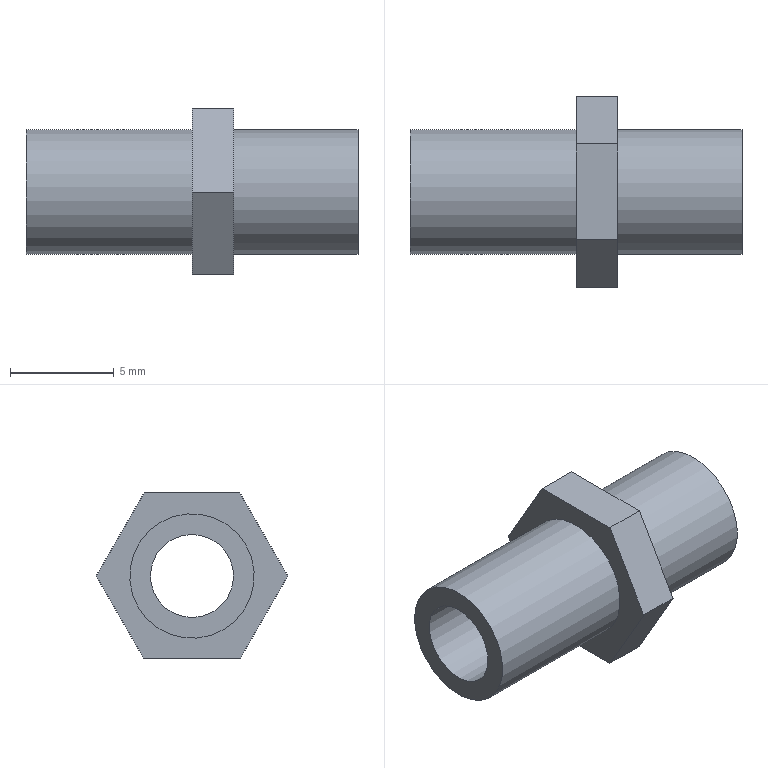Component | NX | PIPE | 1 solid | 13 faces | box 16 x 9.24 x 8 mm | volume 306 mm3 | plane 10 | cylinder 3 | commonest cylinder face diameters 6 x2 4 x1
STEP:
#1=CARTESIAN_POINT('',(0.,0.,0.));
#2=DIRECTION('',(0.,0.,1.));
#3=DIRECTION('',(1.,0.,0.));
#4=AXIS2_PLACEMENT_3D('',#1,#2,#3);
#5=CARTESIAN_POINT('',(-40.,-13.5,42.232));
#6=VERTEX_POINT('',#5);
#7=CARTESIAN_POINT('',(-40.,-14.5,40.5));
#8=DIRECTION('',(1.,0.,0.));
#9=DIRECTION('',(0.,0.5,0.866));
#10=AXIS2_PLACEMENT_3D('',#7,#8,#9);
#11=CIRCLE('',#10,2.);
#12=CARTESIAN_POINT('',(-40.,-14.5,40.5));
#13=DIRECTION('',(-1.,0.,0.));
#14=DIRECTION('',(0.,0.5,0.866));
#15=AXIS2_PLACEMENT_3D('',#12,#13,#14);
#16=PLANE('',#15);
#17=CARTESIAN_POINT('',(2.,-0.));
#18=CARTESIAN_POINT('',(2.,-3.464));
#19=CARTESIAN_POINT('',(-1.,-1.732));
#20=CARTESIAN_POINT('',(-4.,0.));
#21=CARTESIAN_POINT('',(-1.,1.732));
#22=CARTESIAN_POINT('',(2.,3.464));
#23=CARTESIAN_POINT('',(2.,-0.));
#24=(BOUNDED_CURVE()B_SPLINE_CURVE(2,(#17,#18,#19,#20,#21,#22,#23),.UNSPECIFIED.,.T.,.F.)B_SPLINE_CURVE_WITH_KNOTS((1,2,2,2,2,1),(-2.094,0.,2.094,4.189,6.283,8.378),.UNSPECIFIED.)CURVE()GEOMETRIC_REPRESENTATION_ITEM()RATIONAL_B_SPLINE_CURVE((1.,0.5,1.,0.5,1.,0.5,1.))REPRESENTATION_ITEM(''));
#25=(GEOMETRIC_REPRESENTATION_CONTEXT(2)PARAMETRIC_REPRESENTATION_CONTEXT()REPRESENTATION_CONTEXT('',''));
#26=DEFINITIONAL_REPRESENTATION('',(#24),#25);
#27=PCURVE('',#16,#26);
#28=CARTESIAN_POINT('',(-20.,-14.5,40.5));
#29=DIRECTION('',(-1.,0.,0.));
#30=DIRECTION('',(0.,0.5,0.866));
#31=AXIS2_PLACEMENT_3D('',#28,#29,#30);
#32=CYLINDRICAL_SURFACE('',#31,2.);
#33=CARTESIAN_POINT('',(6.283,20.));
#34=DIRECTION('',(-1.,0.));
#35=VECTOR('',#34,1.);
#36=LINE('',#33,#35);
#37=(GEOMETRIC_REPRESENTATION_CONTEXT(2)PARAMETRIC_REPRESENTATION_CONTEXT()REPRESENTATION_CONTEXT('',''));
#38=DEFINITIONAL_REPRESENTATION('',(#36),#37);
#39=PCURVE('',#32,#38);
#40=SURFACE_CURVE('',#11,(#27,#39),.PCURVE_S1.);
#41=EDGE_CURVE('',#6,#6,#40,.T.);
#42=ORIENTED_EDGE('',*,*,#41,.T.);
#43=EDGE_LOOP('',(#42));
#44=FACE_BOUND('',#43,.T.);
#45=CARTESIAN_POINT('',(-40.,-16.,37.902));
#46=VERTEX_POINT('',#45);
#47=CARTESIAN_POINT('',(-40.,-14.5,40.5));
#48=DIRECTION('',(1.,0.,0.));
#49=DIRECTION('',(0.,-0.5,-0.866));
#50=AXIS2_PLACEMENT_3D('',#47,#48,#49);
#51=CIRCLE('',#50,3.);
#52=CARTESIAN_POINT('',(-3.,-0.));
#53=CARTESIAN_POINT('',(-3.,5.196));
#54=CARTESIAN_POINT('',(1.5,2.598));
#55=CARTESIAN_POINT('',(6.,0.));
#56=CARTESIAN_POINT('',(1.5,-2.598));
#57=CARTESIAN_POINT('',(-3.,-5.196));
#58=CARTESIAN_POINT('',(-3.,-0.));
#59=(BOUNDED_CURVE()B_SPLINE_CURVE(2,(#52,#53,#54,#55,#56,#57,#58),.UNSPECIFIED.,.T.,.F.)B_SPLINE_CURVE_WITH_KNOTS((1,2,2,2,2,1),(-2.094,0.,2.094,4.189,6.283,8.378),.UNSPECIFIED.)CURVE()GEOMETRIC_REPRESENTATION_ITEM()RATIONAL_B_SPLINE_CURVE((1.,0.5,1.,0.5,1.,0.5,1.))REPRESENTATION_ITEM(''));
#60=(GEOMETRIC_REPRESENTATION_CONTEXT(2)PARAMETRIC_REPRESENTATION_CONTEXT()REPRESENTATION_CONTEXT('',''));
#61=DEFINITIONAL_REPRESENTATION('',(#59),#60);
#62=PCURVE('',#16,#61);
#63=CARTESIAN_POINT('',(-40.,-14.5,40.5));
#64=DIRECTION('',(1.,0.,0.));
#65=DIRECTION('',(0.,-0.5,-0.866));
#66=AXIS2_PLACEMENT_3D('',#63,#64,#65);
#67=CYLINDRICAL_SURFACE('',#66,3.);
#68=CARTESIAN_POINT('',(0.,0.));
#69=DIRECTION('',(1.,0.));
#70=VECTOR('',#69,1.);
#71=LINE('',#68,#70);
#72=(GEOMETRIC_REPRESENTATION_CONTEXT(2)PARAMETRIC_REPRESENTATION_CONTEXT()REPRESENTATION_CONTEXT('',''));
#73=DEFINITIONAL_REPRESENTATION('',(#71),#72);
#74=PCURVE('',#67,#73);
#75=SURFACE_CURVE('',#51,(#62,#74),.PCURVE_S1.);
#76=EDGE_CURVE('',#46,#46,#75,.T.);
#77=ORIENTED_EDGE('',*,*,#76,.F.);
#78=EDGE_LOOP('',(#77));
#79=FACE_BOUND('',#78,.T.);
#80=ADVANCED_FACE('',(#44,#79),#16,.T.);
#81=CARTESIAN_POINT('',(-32.,-16.,37.902));
#82=VERTEX_POINT('',#81);
#83=CARTESIAN_POINT('',(-32.,-14.5,40.5));
#84=DIRECTION('',(-1.,0.,0.));
#85=DIRECTION('',(0.,-0.5,-0.866));
#86=AXIS2_PLACEMENT_3D('',#83,#84,#85);
#87=CIRCLE('',#86,3.);
#88=CARTESIAN_POINT('',(6.283,8.));
#89=DIRECTION('',(-1.,0.));
#90=VECTOR('',#89,1.);
#91=LINE('',#88,#90);
#92=(GEOMETRIC_REPRESENTATION_CONTEXT(2)PARAMETRIC_REPRESENTATION_CONTEXT()REPRESENTATION_CONTEXT('',''));
#93=DEFINITIONAL_REPRESENTATION('',(#91),#92);
#94=PCURVE('',#67,#93);
#95=CARTESIAN_POINT('',(-32.,-14.5,40.5));
#96=DIRECTION('',(1.,0.,0.));
#97=DIRECTION('',(0.,-0.5,-0.866));
#98=AXIS2_PLACEMENT_3D('',#95,#96,#97);
#99=PLANE('',#98);
#100=CARTESIAN_POINT('',(3.,-0.));
#101=CARTESIAN_POINT('',(3.,-5.196));
#102=CARTESIAN_POINT('',(-1.5,-2.598));
#103=CARTESIAN_POINT('',(-6.,0.));
#104=CARTESIAN_POINT('',(-1.5,2.598));
#105=CARTESIAN_POINT('',(3.,5.196));
#106=CARTESIAN_POINT('',(3.,-0.));
#107=(BOUNDED_CURVE()B_SPLINE_CURVE(2,(#100,#101,#102,#103,#104,#105,#106),.UNSPECIFIED.,.T.,.F.)B_SPLINE_CURVE_WITH_KNOTS((1,2,2,2,2,1),(-2.094,0.,2.094,4.189,6.283,8.378),.UNSPECIFIED.)CURVE()GEOMETRIC_REPRESENTATION_ITEM()RATIONAL_B_SPLINE_CURVE((1.,0.5,1.,0.5,1.,0.5,1.))REPRESENTATION_ITEM(''));
#108=(GEOMETRIC_REPRESENTATION_CONTEXT(2)PARAMETRIC_REPRESENTATION_CONTEXT()REPRESENTATION_CONTEXT('',''));
#109=DEFINITIONAL_REPRESENTATION('',(#107),#108);
#110=PCURVE('',#99,#109);
#111=SURFACE_CURVE('',#87,(#94,#110),.PCURVE_S1.);
#112=EDGE_CURVE('',#82,#82,#111,.T.);
#113=ORIENTED_EDGE('',*,*,#112,.T.);
#114=CARTESIAN_POINT('',(-40.,-16.,37.902));
#115=CARTESIAN_POINT('',(-32.,-16.,37.902));
#116=B_SPLINE_CURVE_WITH_KNOTS('',1,(#114,#115),.UNSPECIFIED.,.F.,.F.,(2,2),(0.,8.),.PIECEWISE_BEZIER_KNOTS.);
#117=CARTESIAN_POINT('',(0.,0.));
#118=DIRECTION('',(0.,1.));
#119=VECTOR('',#118,1.);
#120=LINE('',#117,#119);
#121=(GEOMETRIC_REPRESENTATION_CONTEXT(2)PARAMETRIC_REPRESENTATION_CONTEXT()REPRESENTATION_CONTEXT('',''));
#122=DEFINITIONAL_REPRESENTATION('',(#120),#121);
#123=PCURVE('',#67,#122);
#124=CARTESIAN_POINT('',(6.283,0.));
#125=DIRECTION('',(0.,1.));
#126=VECTOR('',#125,1.);
#127=LINE('',#124,#126);
#128=(GEOMETRIC_REPRESENTATION_CONTEXT(2)PARAMETRIC_REPRESENTATION_CONTEXT()REPRESENTATION_CONTEXT('',''));
#129=DEFINITIONAL_REPRESENTATION('',(#127),#128);
#130=PCURVE('',#67,#129);
#131=SEAM_CURVE('',#116,(#123,#130),.PCURVE_S1.);
#132=EDGE_CURVE('',#46,#82,#131,.T.);
#133=ORIENTED_EDGE('',*,*,#132,.F.);
#134=ORIENTED_EDGE('',*,*,#76,.T.);
#135=ORIENTED_EDGE('',*,*,#132,.T.);
#136=EDGE_LOOP('',(#113,#133,#134,#135));
#137=FACE_BOUND('',#136,.T.);
#138=ADVANCED_FACE('',(#137),#67,.T.);
#139=CARTESIAN_POINT('',(-32.,-12.191,44.5));
#140=VERTEX_POINT('',#139);
#141=CARTESIAN_POINT('',(-32.,-16.809,44.5));
#142=VERTEX_POINT('',#141);
#143=CARTESIAN_POINT('',(-32.,-12.191,44.5));
#144=DIRECTION('',(0.,-1.,-0.));
#145=VECTOR('',#144,1.);
#146=LINE('',#143,#145);
#147=CARTESIAN_POINT('',(-30.,-12.191,44.5));
#148=DIRECTION('',(0.,0.,-1.));
#149=DIRECTION('',(0.,1.,0.));
#150=AXIS2_PLACEMENT_3D('',#147,#148,#149);
#151=PLANE('',#150);
#152=CARTESIAN_POINT('',(0.,-2.));
#153=DIRECTION('',(-1.,0.));
#154=VECTOR('',#153,1.);
#155=LINE('',#152,#154);
#156=(GEOMETRIC_REPRESENTATION_CONTEXT(2)PARAMETRIC_REPRESENTATION_CONTEXT()REPRESENTATION_CONTEXT('',''));
#157=DEFINITIONAL_REPRESENTATION('',(#155),#156);
#158=PCURVE('',#151,#157);
#159=CARTESIAN_POINT('',(-4.619,-0.));
#160=DIRECTION('',(0.5,-0.866));
#161=VECTOR('',#160,1.);
#162=LINE('',#159,#161);
#163=(GEOMETRIC_REPRESENTATION_CONTEXT(2)PARAMETRIC_REPRESENTATION_CONTEXT()REPRESENTATION_CONTEXT('',''));
#164=DEFINITIONAL_REPRESENTATION('',(#162),#163);
#165=PCURVE('',#99,#164);
#166=SURFACE_CURVE('',#146,(#158,#165),.PCURVE_S1.);
#167=EDGE_CURVE('',#140,#142,#166,.T.);
#168=ORIENTED_EDGE('',*,*,#167,.T.);
#169=CARTESIAN_POINT('',(-30.,-16.809,44.5));
#170=VERTEX_POINT('',#169);
#171=CARTESIAN_POINT('',(-30.,-16.809,44.5));
#172=DIRECTION('',(-1.,0.,0.));
#173=VECTOR('',#172,1.);
#174=LINE('',#171,#173);
#175=CARTESIAN_POINT('',(-4.619,0.));
#176=DIRECTION('',(0.,-1.));
#177=VECTOR('',#176,1.);
#178=LINE('',#175,#177);
#179=(GEOMETRIC_REPRESENTATION_CONTEXT(2)PARAMETRIC_REPRESENTATION_CONTEXT()REPRESENTATION_CONTEXT('',''));
#180=DEFINITIONAL_REPRESENTATION('',(#178),#179);
#181=PCURVE('',#151,#180);
#182=CARTESIAN_POINT('',(-30.,-16.809,44.5));
#183=DIRECTION('',(0.,0.866,-0.5));
#184=DIRECTION('',(0.,0.5,0.866));
#185=AXIS2_PLACEMENT_3D('',#182,#183,#184);
#186=PLANE('',#185);
#187=CARTESIAN_POINT('',(0.,0.));
#188=DIRECTION('',(0.,-1.));
#189=VECTOR('',#188,1.);
#190=LINE('',#187,#189);
#191=(GEOMETRIC_REPRESENTATION_CONTEXT(2)PARAMETRIC_REPRESENTATION_CONTEXT()REPRESENTATION_CONTEXT('',''));
#192=DEFINITIONAL_REPRESENTATION('',(#190),#191);
#193=PCURVE('',#186,#192);
#194=SURFACE_CURVE('',#174,(#181,#193),.PCURVE_S1.);
#195=EDGE_CURVE('',#170,#142,#194,.T.);
#196=ORIENTED_EDGE('',*,*,#195,.F.);
#197=CARTESIAN_POINT('',(-30.,-12.191,44.5));
#198=VERTEX_POINT('',#197);
#199=CARTESIAN_POINT('',(-30.,-12.191,44.5));
#200=DIRECTION('',(0.,-1.,-0.));
#201=VECTOR('',#200,1.);
#202=LINE('',#199,#201);
#203=CARTESIAN_POINT('',(0.,0.));
#204=DIRECTION('',(-1.,0.));
#205=VECTOR('',#204,1.);
#206=LINE('',#203,#205);
#207=(GEOMETRIC_REPRESENTATION_CONTEXT(2)PARAMETRIC_REPRESENTATION_CONTEXT()REPRESENTATION_CONTEXT('',''));
#208=DEFINITIONAL_REPRESENTATION('',(#206),#207);
#209=PCURVE('',#151,#208);
#210=CARTESIAN_POINT('',(-30.,-14.5,40.5));
#211=DIRECTION('',(1.,0.,0.));
#212=DIRECTION('',(0.,-0.5,-0.866));
#213=AXIS2_PLACEMENT_3D('',#210,#211,#212);
#214=PLANE('',#213);
#215=CARTESIAN_POINT('',(-4.619,-0.));
#216=DIRECTION('',(0.5,-0.866));
#217=VECTOR('',#216,1.);
#218=LINE('',#215,#217);
#219=(GEOMETRIC_REPRESENTATION_CONTEXT(2)PARAMETRIC_REPRESENTATION_CONTEXT()REPRESENTATION_CONTEXT('',''));
#220=DEFINITIONAL_REPRESENTATION('',(#218),#219);
#221=PCURVE('',#214,#220);
#222=SURFACE_CURVE('',#202,(#209,#221),.PCURVE_S1.);
#223=EDGE_CURVE('',#198,#170,#222,.T.);
#224=ORIENTED_EDGE('',*,*,#223,.F.);
#225=CARTESIAN_POINT('',(-30.,-12.191,44.5));
#226=DIRECTION('',(-1.,0.,0.));
#227=VECTOR('',#226,1.);
#228=LINE('',#225,#227);
#229=CARTESIAN_POINT('',(0.,0.));
#230=DIRECTION('',(0.,-1.));
#231=VECTOR('',#230,1.);
#232=LINE('',#229,#231);
#233=(GEOMETRIC_REPRESENTATION_CONTEXT(2)PARAMETRIC_REPRESENTATION_CONTEXT()REPRESENTATION_CONTEXT('',''));
#234=DEFINITIONAL_REPRESENTATION('',(#232),#233);
#235=PCURVE('',#151,#234);
#236=CARTESIAN_POINT('',(-30.,-9.881,40.5));
#237=DIRECTION('',(0.,-0.866,-0.5));
#238=DIRECTION('',(0.,0.5,-0.866));
#239=AXIS2_PLACEMENT_3D('',#236,#237,#238);
#240=PLANE('',#239);
#241=CARTESIAN_POINT('',(-4.619,0.));
#242=DIRECTION('',(0.,-1.));
#243=VECTOR('',#242,1.);
#244=LINE('',#241,#243);
#245=(GEOMETRIC_REPRESENTATION_CONTEXT(2)PARAMETRIC_REPRESENTATION_CONTEXT()REPRESENTATION_CONTEXT('',''));
#246=DEFINITIONAL_REPRESENTATION('',(#244),#245);
#247=PCURVE('',#240,#246);
#248=SURFACE_CURVE('',#228,(#235,#247),.PCURVE_S1.);
#249=EDGE_CURVE('',#198,#140,#248,.T.);
#250=ORIENTED_EDGE('',*,*,#249,.T.);
#251=EDGE_LOOP('',(#168,#196,#224,#250));
#252=FACE_BOUND('',#251,.T.);
#253=ADVANCED_FACE('',(#252),#151,.F.);
#254=CARTESIAN_POINT('',(-32.,-19.119,40.5));
#255=VERTEX_POINT('',#254);
#256=CARTESIAN_POINT('',(-32.,-16.809,44.5));
#257=DIRECTION('',(0.,-0.5,-0.866));
#258=VECTOR('',#257,1.);
#259=LINE('',#256,#258);
#260=CARTESIAN_POINT('',(0.,-2.));
#261=DIRECTION('',(-1.,0.));
#262=VECTOR('',#261,1.);
#263=LINE('',#260,#262);
#264=(GEOMETRIC_REPRESENTATION_CONTEXT(2)PARAMETRIC_REPRESENTATION_CONTEXT()REPRESENTATION_CONTEXT('',''));
#265=DEFINITIONAL_REPRESENTATION('',(#263),#264);
#266=PCURVE('',#186,#265);
#267=CARTESIAN_POINT('',(-2.309,-4.));
#268=DIRECTION('',(1.,0.));
#269=VECTOR('',#268,1.);
#270=LINE('',#267,#269);
#271=(GEOMETRIC_REPRESENTATION_CONTEXT(2)PARAMETRIC_REPRESENTATION_CONTEXT()REPRESENTATION_CONTEXT('',''));
#272=DEFINITIONAL_REPRESENTATION('',(#270),#271);
#273=PCURVE('',#99,#272);
#274=SURFACE_CURVE('',#259,(#266,#273),.PCURVE_S1.);
#275=EDGE_CURVE('',#142,#255,#274,.T.);
#276=ORIENTED_EDGE('',*,*,#275,.T.);
#277=CARTESIAN_POINT('',(-30.,-19.119,40.5));
#278=VERTEX_POINT('',#277);
#279=CARTESIAN_POINT('',(-30.,-19.119,40.5));
#280=DIRECTION('',(-1.,0.,0.));
#281=VECTOR('',#280,1.);
#282=LINE('',#279,#281);
#283=CARTESIAN_POINT('',(-4.619,0.));
#284=DIRECTION('',(0.,-1.));
#285=VECTOR('',#284,1.);
#286=LINE('',#283,#285);
#287=(GEOMETRIC_REPRESENTATION_CONTEXT(2)PARAMETRIC_REPRESENTATION_CONTEXT()REPRESENTATION_CONTEXT('',''));
#288=DEFINITIONAL_REPRESENTATION('',(#286),#287);
#289=PCURVE('',#186,#288);
#290=CARTESIAN_POINT('',(-30.,-19.119,40.5));
#291=DIRECTION('',(0.,0.866,0.5));
#292=DIRECTION('',(0.,-0.5,0.866));
#293=AXIS2_PLACEMENT_3D('',#290,#291,#292);
#294=PLANE('',#293);
#295=CARTESIAN_POINT('',(0.,0.));
#296=DIRECTION('',(0.,-1.));
#297=VECTOR('',#296,1.);
#298=LINE('',#295,#297);
#299=(GEOMETRIC_REPRESENTATION_CONTEXT(2)PARAMETRIC_REPRESENTATION_CONTEXT()REPRESENTATION_CONTEXT('',''));
#300=DEFINITIONAL_REPRESENTATION('',(#298),#299);
#301=PCURVE('',#294,#300);
#302=SURFACE_CURVE('',#282,(#289,#301),.PCURVE_S1.);
#303=EDGE_CURVE('',#278,#255,#302,.T.);
#304=ORIENTED_EDGE('',*,*,#303,.F.);
#305=CARTESIAN_POINT('',(-30.,-16.809,44.5));
#306=DIRECTION('',(0.,-0.5,-0.866));
#307=VECTOR('',#306,1.);
#308=LINE('',#305,#307);
#309=CARTESIAN_POINT('',(0.,0.));
#310=DIRECTION('',(-1.,0.));
#311=VECTOR('',#310,1.);
#312=LINE('',#309,#311);
#313=(GEOMETRIC_REPRESENTATION_CONTEXT(2)PARAMETRIC_REPRESENTATION_CONTEXT()REPRESENTATION_CONTEXT('',''));
#314=DEFINITIONAL_REPRESENTATION('',(#312),#313);
#315=PCURVE('',#186,#314);
#316=CARTESIAN_POINT('',(-2.309,-4.));
#317=DIRECTION('',(1.,0.));
#318=VECTOR('',#317,1.);
#319=LINE('',#316,#318);
#320=(GEOMETRIC_REPRESENTATION_CONTEXT(2)PARAMETRIC_REPRESENTATION_CONTEXT()REPRESENTATION_CONTEXT('',''));
#321=DEFINITIONAL_REPRESENTATION('',(#319),#320);
#322=PCURVE('',#214,#321);
#323=SURFACE_CURVE('',#308,(#315,#322),.PCURVE_S1.);
#324=EDGE_CURVE('',#170,#278,#323,.T.);
#325=ORIENTED_EDGE('',*,*,#324,.F.);
#326=ORIENTED_EDGE('',*,*,#195,.T.);
#327=EDGE_LOOP('',(#276,#304,#325,#326));
#328=FACE_BOUND('',#327,.T.);
#329=ADVANCED_FACE('',(#328),#186,.F.);
#330=CARTESIAN_POINT('',(-32.,-16.809,36.5));
#331=VERTEX_POINT('',#330);
#332=CARTESIAN_POINT('',(-32.,-19.119,40.5));
#333=DIRECTION('',(0.,0.5,-0.866));
#334=VECTOR('',#333,1.);
#335=LINE('',#332,#334);
#336=CARTESIAN_POINT('',(0.,-2.));
#337=DIRECTION('',(-1.,0.));
#338=VECTOR('',#337,1.);
#339=LINE('',#336,#338);
#340=(GEOMETRIC_REPRESENTATION_CONTEXT(2)PARAMETRIC_REPRESENTATION_CONTEXT()REPRESENTATION_CONTEXT('',''));
#341=DEFINITIONAL_REPRESENTATION('',(#339),#340);
#342=PCURVE('',#294,#341);
#343=CARTESIAN_POINT('',(2.309,-4.));
#344=DIRECTION('',(0.5,0.866));
#345=VECTOR('',#344,1.);
#346=LINE('',#343,#345);
#347=(GEOMETRIC_REPRESENTATION_CONTEXT(2)PARAMETRIC_REPRESENTATION_CONTEXT()REPRESENTATION_CONTEXT('',''));
#348=DEFINITIONAL_REPRESENTATION('',(#346),#347);
#349=PCURVE('',#99,#348);
#350=SURFACE_CURVE('',#335,(#342,#349),.PCURVE_S1.);
#351=EDGE_CURVE('',#255,#331,#350,.T.);
#352=ORIENTED_EDGE('',*,*,#351,.T.);
#353=CARTESIAN_POINT('',(-30.,-16.809,36.5));
#354=VERTEX_POINT('',#353);
#355=CARTESIAN_POINT('',(-30.,-16.809,36.5));
#356=DIRECTION('',(-1.,0.,0.));
#357=VECTOR('',#356,1.);
#358=LINE('',#355,#357);
#359=CARTESIAN_POINT('',(-4.619,0.));
#360=DIRECTION('',(0.,-1.));
#361=VECTOR('',#360,1.);
#362=LINE('',#359,#361);
#363=(GEOMETRIC_REPRESENTATION_CONTEXT(2)PARAMETRIC_REPRESENTATION_CONTEXT()REPRESENTATION_CONTEXT('',''));
#364=DEFINITIONAL_REPRESENTATION('',(#362),#363);
#365=PCURVE('',#294,#364);
#366=CARTESIAN_POINT('',(-30.,-16.809,36.5));
#367=DIRECTION('',(0.,-0.,1.));
#368=DIRECTION('',(0.,-1.,-0.));
#369=AXIS2_PLACEMENT_3D('',#366,#367,#368);
#370=PLANE('',#369);
#371=CARTESIAN_POINT('',(0.,0.));
#372=DIRECTION('',(0.,-1.));
#373=VECTOR('',#372,1.);
#374=LINE('',#371,#373);
#375=(GEOMETRIC_REPRESENTATION_CONTEXT(2)PARAMETRIC_REPRESENTATION_CONTEXT()REPRESENTATION_CONTEXT('',''));
#376=DEFINITIONAL_REPRESENTATION('',(#374),#375);
#377=PCURVE('',#370,#376);
#378=SURFACE_CURVE('',#358,(#365,#377),.PCURVE_S1.);
#379=EDGE_CURVE('',#354,#331,#378,.T.);
#380=ORIENTED_EDGE('',*,*,#379,.F.);
#381=CARTESIAN_POINT('',(-30.,-19.119,40.5));
#382=DIRECTION('',(0.,0.5,-0.866));
#383=VECTOR('',#382,1.);
#384=LINE('',#381,#383);
#385=CARTESIAN_POINT('',(0.,0.));
#386=DIRECTION('',(-1.,0.));
#387=VECTOR('',#386,1.);
#388=LINE('',#385,#387);
#389=(GEOMETRIC_REPRESENTATION_CONTEXT(2)PARAMETRIC_REPRESENTATION_CONTEXT()REPRESENTATION_CONTEXT('',''));
#390=DEFINITIONAL_REPRESENTATION('',(#388),#389);
#391=PCURVE('',#294,#390);
#392=CARTESIAN_POINT('',(2.309,-4.));
#393=DIRECTION('',(0.5,0.866));
#394=VECTOR('',#393,1.);
#395=LINE('',#392,#394);
#396=(GEOMETRIC_REPRESENTATION_CONTEXT(2)PARAMETRIC_REPRESENTATION_CONTEXT()REPRESENTATION_CONTEXT('',''));
#397=DEFINITIONAL_REPRESENTATION('',(#395),#396);
#398=PCURVE('',#214,#397);
#399=SURFACE_CURVE('',#384,(#391,#398),.PCURVE_S1.);
#400=EDGE_CURVE('',#278,#354,#399,.T.);
#401=ORIENTED_EDGE('',*,*,#400,.F.);
#402=ORIENTED_EDGE('',*,*,#303,.T.);
#403=EDGE_LOOP('',(#352,#380,#401,#402));
#404=FACE_BOUND('',#403,.T.);
#405=ADVANCED_FACE('',(#404),#294,.F.);
#406=CARTESIAN_POINT('',(-32.,-12.191,36.5));
#407=VERTEX_POINT('',#406);
#408=CARTESIAN_POINT('',(-32.,-16.809,36.5));
#409=DIRECTION('',(0.,1.,0.));
#410=VECTOR('',#409,1.);
#411=LINE('',#408,#410);
#412=CARTESIAN_POINT('',(0.,-2.));
#413=DIRECTION('',(-1.,0.));
#414=VECTOR('',#413,1.);
#415=LINE('',#412,#414);
#416=(GEOMETRIC_REPRESENTATION_CONTEXT(2)PARAMETRIC_REPRESENTATION_CONTEXT()REPRESENTATION_CONTEXT('',''));
#417=DEFINITIONAL_REPRESENTATION('',(#415),#416);
#418=PCURVE('',#370,#417);
#419=CARTESIAN_POINT('',(4.619,0.));
#420=DIRECTION('',(-0.5,0.866));
#421=VECTOR('',#420,1.);
#422=LINE('',#419,#421);
#423=(GEOMETRIC_REPRESENTATION_CONTEXT(2)PARAMETRIC_REPRESENTATION_CONTEXT()REPRESENTATION_CONTEXT('',''));
#424=DEFINITIONAL_REPRESENTATION('',(#422),#423);
#425=PCURVE('',#99,#424);
#426=SURFACE_CURVE('',#411,(#418,#425),.PCURVE_S1.);
#427=EDGE_CURVE('',#331,#407,#426,.T.);
#428=ORIENTED_EDGE('',*,*,#427,.T.);
#429=CARTESIAN_POINT('',(-30.,-12.191,36.5));
#430=VERTEX_POINT('',#429);
#431=CARTESIAN_POINT('',(-30.,-12.191,36.5));
#432=DIRECTION('',(-1.,0.,0.));
#433=VECTOR('',#432,1.);
#434=LINE('',#431,#433);
#435=CARTESIAN_POINT('',(-4.619,0.));
#436=DIRECTION('',(0.,-1.));
#437=VECTOR('',#436,1.);
#438=LINE('',#435,#437);
#439=(GEOMETRIC_REPRESENTATION_CONTEXT(2)PARAMETRIC_REPRESENTATION_CONTEXT()REPRESENTATION_CONTEXT('',''));
#440=DEFINITIONAL_REPRESENTATION('',(#438),#439);
#441=PCURVE('',#370,#440);
#442=CARTESIAN_POINT('',(-30.,-12.191,36.5));
#443=DIRECTION('',(0.,-0.866,0.5));
#444=DIRECTION('',(0.,-0.5,-0.866));
#445=AXIS2_PLACEMENT_3D('',#442,#443,#444);
#446=PLANE('',#445);
#447=CARTESIAN_POINT('',(0.,0.));
#448=DIRECTION('',(0.,-1.));
#449=VECTOR('',#448,1.);
#450=LINE('',#447,#449);
#451=(GEOMETRIC_REPRESENTATION_CONTEXT(2)PARAMETRIC_REPRESENTATION_CONTEXT()REPRESENTATION_CONTEXT('',''));
#452=DEFINITIONAL_REPRESENTATION('',(#450),#451);
#453=PCURVE('',#446,#452);
#454=SURFACE_CURVE('',#434,(#441,#453),.PCURVE_S1.);
#455=EDGE_CURVE('',#430,#407,#454,.T.);
#456=ORIENTED_EDGE('',*,*,#455,.F.);
#457=CARTESIAN_POINT('',(-30.,-16.809,36.5));
#458=DIRECTION('',(0.,1.,0.));
#459=VECTOR('',#458,1.);
#460=LINE('',#457,#459);
#461=CARTESIAN_POINT('',(0.,0.));
#462=DIRECTION('',(-1.,0.));
#463=VECTOR('',#462,1.);
#464=LINE('',#461,#463);
#465=(GEOMETRIC_REPRESENTATION_CONTEXT(2)PARAMETRIC_REPRESENTATION_CONTEXT()REPRESENTATION_CONTEXT('',''));
#466=DEFINITIONAL_REPRESENTATION('',(#464),#465);
#467=PCURVE('',#370,#466);
#468=CARTESIAN_POINT('',(4.619,0.));
#469=DIRECTION('',(-0.5,0.866));
#470=VECTOR('',#469,1.);
#471=LINE('',#468,#470);
#472=(GEOMETRIC_REPRESENTATION_CONTEXT(2)PARAMETRIC_REPRESENTATION_CONTEXT()REPRESENTATION_CONTEXT('',''));
#473=DEFINITIONAL_REPRESENTATION('',(#471),#472);
#474=PCURVE('',#214,#473);
#475=SURFACE_CURVE('',#460,(#467,#474),.PCURVE_S1.);
#476=EDGE_CURVE('',#354,#430,#475,.T.);
#477=ORIENTED_EDGE('',*,*,#476,.F.);
#478=ORIENTED_EDGE('',*,*,#379,.T.);
#479=EDGE_LOOP('',(#428,#456,#477,#478));
#480=FACE_BOUND('',#479,.T.);
#481=ADVANCED_FACE('',(#480),#370,.F.);
#482=CARTESIAN_POINT('',(-32.,-9.881,40.5));
#483=VERTEX_POINT('',#482);
#484=CARTESIAN_POINT('',(-32.,-12.191,36.5));
#485=DIRECTION('',(0.,0.5,0.866));
#486=VECTOR('',#485,1.);
#487=LINE('',#484,#486);
#488=CARTESIAN_POINT('',(0.,-2.));
#489=DIRECTION('',(-1.,0.));
#490=VECTOR('',#489,1.);
#491=LINE('',#488,#490);
#492=(GEOMETRIC_REPRESENTATION_CONTEXT(2)PARAMETRIC_REPRESENTATION_CONTEXT()REPRESENTATION_CONTEXT('',''));
#493=DEFINITIONAL_REPRESENTATION('',(#491),#492);
#494=PCURVE('',#446,#493);
#495=CARTESIAN_POINT('',(2.309,4.));
#496=DIRECTION('',(-1.,0.));
#497=VECTOR('',#496,1.);
#498=LINE('',#495,#497);
#499=(GEOMETRIC_REPRESENTATION_CONTEXT(2)PARAMETRIC_REPRESENTATION_CONTEXT()REPRESENTATION_CONTEXT('',''));
#500=DEFINITIONAL_REPRESENTATION('',(#498),#499);
#501=PCURVE('',#99,#500);
#502=SURFACE_CURVE('',#487,(#494,#501),.PCURVE_S1.);
#503=EDGE_CURVE('',#407,#483,#502,.T.);
#504=ORIENTED_EDGE('',*,*,#503,.T.);
#505=CARTESIAN_POINT('',(-30.,-9.881,40.5));
#506=VERTEX_POINT('',#505);
#507=CARTESIAN_POINT('',(-30.,-9.881,40.5));
#508=DIRECTION('',(-1.,0.,0.));
#509=VECTOR('',#508,1.);
#510=LINE('',#507,#509);
#511=CARTESIAN_POINT('',(-4.619,0.));
#512=DIRECTION('',(0.,-1.));
#513=VECTOR('',#512,1.);
#514=LINE('',#511,#513);
#515=(GEOMETRIC_REPRESENTATION_CONTEXT(2)PARAMETRIC_REPRESENTATION_CONTEXT()REPRESENTATION_CONTEXT('',''));
#516=DEFINITIONAL_REPRESENTATION('',(#514),#515);
#517=PCURVE('',#446,#516);
#518=CARTESIAN_POINT('',(0.,0.));
#519=DIRECTION('',(0.,-1.));
#520=VECTOR('',#519,1.);
#521=LINE('',#518,#520);
#522=(GEOMETRIC_REPRESENTATION_CONTEXT(2)PARAMETRIC_REPRESENTATION_CONTEXT()REPRESENTATION_CONTEXT('',''));
#523=DEFINITIONAL_REPRESENTATION('',(#521),#522);
#524=PCURVE('',#240,#523);
#525=SURFACE_CURVE('',#510,(#517,#524),.PCURVE_S1.);
#526=EDGE_CURVE('',#506,#483,#525,.T.);
#527=ORIENTED_EDGE('',*,*,#526,.F.);
#528=CARTESIAN_POINT('',(-30.,-12.191,36.5));
#529=DIRECTION('',(0.,0.5,0.866));
#530=VECTOR('',#529,1.);
#531=LINE('',#528,#530);
#532=CARTESIAN_POINT('',(0.,0.));
#533=DIRECTION('',(-1.,0.));
#534=VECTOR('',#533,1.);
#535=LINE('',#532,#534);
#536=(GEOMETRIC_REPRESENTATION_CONTEXT(2)PARAMETRIC_REPRESENTATION_CONTEXT()REPRESENTATION_CONTEXT('',''));
#537=DEFINITIONAL_REPRESENTATION('',(#535),#536);
#538=PCURVE('',#446,#537);
#539=CARTESIAN_POINT('',(2.309,4.));
#540=DIRECTION('',(-1.,0.));
#541=VECTOR('',#540,1.);
#542=LINE('',#539,#541);
#543=(GEOMETRIC_REPRESENTATION_CONTEXT(2)PARAMETRIC_REPRESENTATION_CONTEXT()REPRESENTATION_CONTEXT('',''));
#544=DEFINITIONAL_REPRESENTATION('',(#542),#543);
#545=PCURVE('',#214,#544);
#546=SURFACE_CURVE('',#531,(#538,#545),.PCURVE_S1.);
#547=EDGE_CURVE('',#430,#506,#546,.T.);
#548=ORIENTED_EDGE('',*,*,#547,.F.);
#549=ORIENTED_EDGE('',*,*,#455,.T.);
#550=EDGE_LOOP('',(#504,#527,#548,#549));
#551=FACE_BOUND('',#550,.T.);
#552=ADVANCED_FACE('',(#551),#446,.F.);
#553=CARTESIAN_POINT('',(-32.,-9.881,40.5));
#554=DIRECTION('',(0.,-0.5,0.866));
#555=VECTOR('',#554,1.);
#556=LINE('',#553,#555);
#557=CARTESIAN_POINT('',(0.,-2.));
#558=DIRECTION('',(-1.,0.));
#559=VECTOR('',#558,1.);
#560=LINE('',#557,#559);
#561=(GEOMETRIC_REPRESENTATION_CONTEXT(2)PARAMETRIC_REPRESENTATION_CONTEXT()REPRESENTATION_CONTEXT('',''));
#562=DEFINITIONAL_REPRESENTATION('',(#560),#561);
#563=PCURVE('',#240,#562);
#564=CARTESIAN_POINT('',(-2.309,4.));
#565=DIRECTION('',(-0.5,-0.866));
#566=VECTOR('',#565,1.);
#567=LINE('',#564,#566);
#568=(GEOMETRIC_REPRESENTATION_CONTEXT(2)PARAMETRIC_REPRESENTATION_CONTEXT()REPRESENTATION_CONTEXT('',''));
#569=DEFINITIONAL_REPRESENTATION('',(#567),#568);
#570=PCURVE('',#99,#569);
#571=SURFACE_CURVE('',#556,(#563,#570),.PCURVE_S1.);
#572=EDGE_CURVE('',#483,#140,#571,.T.);
#573=ORIENTED_EDGE('',*,*,#572,.T.);
#574=ORIENTED_EDGE('',*,*,#249,.F.);
#575=CARTESIAN_POINT('',(-30.,-9.881,40.5));
#576=DIRECTION('',(0.,-0.5,0.866));
#577=VECTOR('',#576,1.);
#578=LINE('',#575,#577);
#579=CARTESIAN_POINT('',(0.,0.));
#580=DIRECTION('',(-1.,0.));
#581=VECTOR('',#580,1.);
#582=LINE('',#579,#581);
#583=(GEOMETRIC_REPRESENTATION_CONTEXT(2)PARAMETRIC_REPRESENTATION_CONTEXT()REPRESENTATION_CONTEXT('',''));
#584=DEFINITIONAL_REPRESENTATION('',(#582),#583);
#585=PCURVE('',#240,#584);
#586=CARTESIAN_POINT('',(-2.309,4.));
#587=DIRECTION('',(-0.5,-0.866));
#588=VECTOR('',#587,1.);
#589=LINE('',#586,#588);
#590=(GEOMETRIC_REPRESENTATION_CONTEXT(2)PARAMETRIC_REPRESENTATION_CONTEXT()REPRESENTATION_CONTEXT('',''));
#591=DEFINITIONAL_REPRESENTATION('',(#589),#590);
#592=PCURVE('',#214,#591);
#593=SURFACE_CURVE('',#578,(#585,#592),.PCURVE_S1.);
#594=EDGE_CURVE('',#506,#198,#593,.T.);
#595=ORIENTED_EDGE('',*,*,#594,.F.);
#596=ORIENTED_EDGE('',*,*,#526,.T.);
#597=EDGE_LOOP('',(#573,#574,#595,#596));
#598=FACE_BOUND('',#597,.T.);
#599=ADVANCED_FACE('',(#598),#240,.F.);
#600=CARTESIAN_POINT('',(-30.,-13.,37.902));
#601=VERTEX_POINT('',#600);
#602=CARTESIAN_POINT('',(-30.,-14.5,40.5));
#603=DIRECTION('',(1.,0.,0.));
#604=DIRECTION('',(0.,0.5,-0.866));
#605=AXIS2_PLACEMENT_3D('',#602,#603,#604);
#606=CIRCLE('',#605,3.);
#607=CARTESIAN_POINT('',(0.,0.));
#608=DIRECTION('',(0.5,0.866));
#609=AXIS2_PLACEMENT_2D('',#607,#608);
#610=CIRCLE('',#609,3.);
#611=(GEOMETRIC_REPRESENTATION_CONTEXT(2)PARAMETRIC_REPRESENTATION_CONTEXT()REPRESENTATION_CONTEXT('',''));
#612=DEFINITIONAL_REPRESENTATION('',(#610),#611);
#613=PCURVE('',#214,#612);
#614=CARTESIAN_POINT('',(-24.,-14.5,40.5));
#615=DIRECTION('',(-1.,0.,0.));
#616=DIRECTION('',(0.,0.5,0.866));
#617=AXIS2_PLACEMENT_3D('',#614,#615,#616);
#618=CYLINDRICAL_SURFACE('',#617,3.);
#619=CARTESIAN_POINT('',(8.378,6.));
#620=DIRECTION('',(-1.,0.));
#621=VECTOR('',#620,1.);
#622=LINE('',#619,#621);
#623=(GEOMETRIC_REPRESENTATION_CONTEXT(2)PARAMETRIC_REPRESENTATION_CONTEXT()REPRESENTATION_CONTEXT('',''));
#624=DEFINITIONAL_REPRESENTATION('',(#622),#623);
#625=PCURVE('',#618,#624);
#626=SURFACE_CURVE('',#606,(#613,#625),.PCURVE_S1.);
#627=EDGE_CURVE('',#601,#601,#626,.T.);
#628=ORIENTED_EDGE('',*,*,#627,.F.);
#629=EDGE_LOOP('',(#628));
#630=FACE_BOUND('',#629,.T.);
#631=ORIENTED_EDGE('',*,*,#223,.T.);
#632=ORIENTED_EDGE('',*,*,#324,.T.);
#633=ORIENTED_EDGE('',*,*,#400,.T.);
#634=ORIENTED_EDGE('',*,*,#476,.T.);
#635=ORIENTED_EDGE('',*,*,#547,.T.);
#636=ORIENTED_EDGE('',*,*,#594,.T.);
#637=EDGE_LOOP('',(#631,#632,#633,#634,#635,#636));
#638=FACE_BOUND('',#637,.T.);
#639=ADVANCED_FACE('',(#630,#638),#214,.T.);
#640=ORIENTED_EDGE('',*,*,#112,.F.);
#641=EDGE_LOOP('',(#640));
#642=FACE_BOUND('',#641,.T.);
#643=ORIENTED_EDGE('',*,*,#167,.F.);
#644=ORIENTED_EDGE('',*,*,#572,.F.);
#645=ORIENTED_EDGE('',*,*,#503,.F.);
#646=ORIENTED_EDGE('',*,*,#427,.F.);
#647=ORIENTED_EDGE('',*,*,#351,.F.);
#648=ORIENTED_EDGE('',*,*,#275,.F.);
#649=EDGE_LOOP('',(#643,#644,#645,#646,#647,#648));
#650=FACE_BOUND('',#649,.T.);
#651=ADVANCED_FACE('',(#642,#650),#99,.F.);
#652=CARTESIAN_POINT('',(-24.,-13.,37.902));
#653=VERTEX_POINT('',#652);
#654=CARTESIAN_POINT('',(-24.,-14.5,40.5));
#655=DIRECTION('',(1.,0.,0.));
#656=DIRECTION('',(0.,0.5,-0.866));
#657=AXIS2_PLACEMENT_3D('',#654,#655,#656);
#658=CIRCLE('',#657,3.);
#659=CARTESIAN_POINT('',(8.378,0.));
#660=DIRECTION('',(-1.,0.));
#661=VECTOR('',#660,1.);
#662=LINE('',#659,#661);
#663=(GEOMETRIC_REPRESENTATION_CONTEXT(2)PARAMETRIC_REPRESENTATION_CONTEXT()REPRESENTATION_CONTEXT('',''));
#664=DEFINITIONAL_REPRESENTATION('',(#662),#663);
#665=PCURVE('',#618,#664);
#666=CARTESIAN_POINT('',(-24.,-14.5,40.5));
#667=DIRECTION('',(1.,0.,0.));
#668=DIRECTION('',(0.,-0.5,-0.866));
#669=AXIS2_PLACEMENT_3D('',#666,#667,#668);
#670=PLANE('',#669);
#671=CARTESIAN_POINT('',(0.,0.));
#672=DIRECTION('',(0.5,0.866));
#673=AXIS2_PLACEMENT_2D('',#671,#672);
#674=CIRCLE('',#673,3.);
#675=(GEOMETRIC_REPRESENTATION_CONTEXT(2)PARAMETRIC_REPRESENTATION_CONTEXT()REPRESENTATION_CONTEXT('',''));
#676=DEFINITIONAL_REPRESENTATION('',(#674),#675);
#677=PCURVE('',#670,#676);
#678=SURFACE_CURVE('',#658,(#665,#677),.PCURVE_S1.);
#679=EDGE_CURVE('',#653,#653,#678,.T.);
#680=ORIENTED_EDGE('',*,*,#679,.F.);
#681=CARTESIAN_POINT('',(-24.,-13.,37.902));
#682=CARTESIAN_POINT('',(-30.,-13.,37.902));
#683=B_SPLINE_CURVE_WITH_KNOTS('',1,(#681,#682),.UNSPECIFIED.,.F.,.F.,(2,2),(0.,6.),.PIECEWISE_BEZIER_KNOTS.);
#684=CARTESIAN_POINT('',(8.378,0.));
#685=DIRECTION('',(0.,1.));
#686=VECTOR('',#685,1.);
#687=LINE('',#684,#686);
#688=(GEOMETRIC_REPRESENTATION_CONTEXT(2)PARAMETRIC_REPRESENTATION_CONTEXT()REPRESENTATION_CONTEXT('',''));
#689=DEFINITIONAL_REPRESENTATION('',(#687),#688);
#690=PCURVE('',#618,#689);
#691=CARTESIAN_POINT('',(2.094,0.));
#692=DIRECTION('',(0.,1.));
#693=VECTOR('',#692,1.);
#694=LINE('',#691,#693);
#695=(GEOMETRIC_REPRESENTATION_CONTEXT(2)PARAMETRIC_REPRESENTATION_CONTEXT()REPRESENTATION_CONTEXT('',''));
#696=DEFINITIONAL_REPRESENTATION('',(#694),#695);
#697=PCURVE('',#618,#696);
#698=SEAM_CURVE('',#683,(#690,#697),.PCURVE_S1.);
#699=EDGE_CURVE('',#653,#601,#698,.T.);
#700=ORIENTED_EDGE('',*,*,#699,.T.);
#701=ORIENTED_EDGE('',*,*,#627,.T.);
#702=ORIENTED_EDGE('',*,*,#699,.F.);
#703=EDGE_LOOP('',(#680,#700,#701,#702));
#704=FACE_BOUND('',#703,.T.);
#705=ADVANCED_FACE('',(#704),#618,.T.);
#706=CARTESIAN_POINT('',(-24.,-15.5,38.768));
#707=VERTEX_POINT('',#706);
#708=CARTESIAN_POINT('',(-24.,-13.5,42.232));
#709=VERTEX_POINT('',#708);
#710=CARTESIAN_POINT('',(-24.,-14.5,40.5));
#711=DIRECTION('',(-1.,0.,0.));
#712=DIRECTION('',(0.,-0.5,-0.866));
#713=AXIS2_PLACEMENT_3D('',#710,#711,#712);
#714=CIRCLE('',#713,2.);
#715=CARTESIAN_POINT('',(2.,0.));
#716=CARTESIAN_POINT('',(2.,-3.464));
#717=CARTESIAN_POINT('',(-1.,-1.732));
#718=CARTESIAN_POINT('',(-4.,-0.));
#719=CARTESIAN_POINT('',(-1.,1.732));
#720=CARTESIAN_POINT('',(2.,3.464));
#721=CARTESIAN_POINT('',(2.,0.));
#722=(BOUNDED_CURVE()B_SPLINE_CURVE(2,(#715,#716,#717,#718,#719,#720,#721),.UNSPECIFIED.,.T.,.F.)B_SPLINE_CURVE_WITH_KNOTS((1,2,2,2,2,1),(-2.094,0.,2.094,4.189,6.283,8.378),.UNSPECIFIED.)CURVE()GEOMETRIC_REPRESENTATION_ITEM()RATIONAL_B_SPLINE_CURVE((1.,0.5,1.,0.5,1.,0.5,1.))REPRESENTATION_ITEM(''));
#723=(GEOMETRIC_REPRESENTATION_CONTEXT(2)PARAMETRIC_REPRESENTATION_CONTEXT()REPRESENTATION_CONTEXT('',''));
#724=DEFINITIONAL_REPRESENTATION('',(#722),#723);
#725=PCURVE('',#670,#724);
#726=CARTESIAN_POINT('',(3.142,4.));
#727=DIRECTION('',(1.,0.));
#728=VECTOR('',#727,1.);
#729=LINE('',#726,#728);
#730=(GEOMETRIC_REPRESENTATION_CONTEXT(2)PARAMETRIC_REPRESENTATION_CONTEXT()REPRESENTATION_CONTEXT('',''));
#731=DEFINITIONAL_REPRESENTATION('',(#729),#730);
#732=PCURVE('',#32,#731);
#733=SURFACE_CURVE('',#714,(#725,#732),.PCURVE_S1.);
#734=EDGE_CURVE('',#707,#709,#733,.T.);
#735=ORIENTED_EDGE('',*,*,#734,.T.);
#736=CARTESIAN_POINT('',(-24.,-14.5,40.5));
#737=DIRECTION('',(-1.,0.,0.));
#738=DIRECTION('',(0.,-0.5,-0.866));
#739=AXIS2_PLACEMENT_3D('',#736,#737,#738);
#740=CIRCLE('',#739,2.);
#741=CARTESIAN_POINT('',(2.,0.));
#742=CARTESIAN_POINT('',(2.,-3.464));
#743=CARTESIAN_POINT('',(-1.,-1.732));
#744=CARTESIAN_POINT('',(-4.,-0.));
#745=CARTESIAN_POINT('',(-1.,1.732));
#746=CARTESIAN_POINT('',(2.,3.464));
#747=CARTESIAN_POINT('',(2.,0.));
#748=(BOUNDED_CURVE()B_SPLINE_CURVE(2,(#741,#742,#743,#744,#745,#746,#747),.UNSPECIFIED.,.T.,.F.)B_SPLINE_CURVE_WITH_KNOTS((1,2,2,2,2,1),(-2.094,0.,2.094,4.189,6.283,8.378),.UNSPECIFIED.)CURVE()GEOMETRIC_REPRESENTATION_ITEM()RATIONAL_B_SPLINE_CURVE((1.,0.5,1.,0.5,1.,0.5,1.))REPRESENTATION_ITEM(''));
#749=(GEOMETRIC_REPRESENTATION_CONTEXT(2)PARAMETRIC_REPRESENTATION_CONTEXT()REPRESENTATION_CONTEXT('',''));
#750=DEFINITIONAL_REPRESENTATION('',(#748),#749);
#751=PCURVE('',#670,#750);
#752=CARTESIAN_POINT('',(-3.142,4.));
#753=DIRECTION('',(1.,0.));
#754=VECTOR('',#753,1.);
#755=LINE('',#752,#754);
#756=(GEOMETRIC_REPRESENTATION_CONTEXT(2)PARAMETRIC_REPRESENTATION_CONTEXT()REPRESENTATION_CONTEXT('',''));
#757=DEFINITIONAL_REPRESENTATION('',(#755),#756);
#758=PCURVE('',#32,#757);
#759=SURFACE_CURVE('',#740,(#751,#758),.PCURVE_S1.);
#760=EDGE_CURVE('',#709,#707,#759,.T.);
#761=ORIENTED_EDGE('',*,*,#760,.T.);
#762=EDGE_LOOP('',(#735,#761));
#763=FACE_BOUND('',#762,.T.);
#764=ORIENTED_EDGE('',*,*,#679,.T.);
#765=EDGE_LOOP('',(#764));
#766=FACE_BOUND('',#765,.T.);
#767=ADVANCED_FACE('',(#763,#766),#670,.T.);
#768=ORIENTED_EDGE('',*,*,#41,.T.);
#769=CARTESIAN_POINT('',(-24.,-13.5,42.232));
#770=CARTESIAN_POINT('',(-40.,-13.5,42.232));
#771=B_SPLINE_CURVE_WITH_KNOTS('',1,(#769,#770),.UNSPECIFIED.,.F.,.F.,(2,2),(4.,20.),.PIECEWISE_BEZIER_KNOTS.);
#772=CARTESIAN_POINT('',(0.,0.));
#773=DIRECTION('',(0.,1.));
#774=VECTOR('',#773,1.);
#775=LINE('',#772,#774);
#776=(GEOMETRIC_REPRESENTATION_CONTEXT(2)PARAMETRIC_REPRESENTATION_CONTEXT()REPRESENTATION_CONTEXT('',''));
#777=DEFINITIONAL_REPRESENTATION('',(#775),#776);
#778=PCURVE('',#32,#777);
#779=CARTESIAN_POINT('',(6.283,0.));
#780=DIRECTION('',(0.,1.));
#781=VECTOR('',#780,1.);
#782=LINE('',#779,#781);
#783=(GEOMETRIC_REPRESENTATION_CONTEXT(2)PARAMETRIC_REPRESENTATION_CONTEXT()REPRESENTATION_CONTEXT('',''));
#784=DEFINITIONAL_REPRESENTATION('',(#782),#783);
#785=PCURVE('',#32,#784);
#786=SEAM_CURVE('',#771,(#778,#785),.PCURVE_S1.);
#787=EDGE_CURVE('',#709,#6,#786,.T.);
#788=ORIENTED_EDGE('',*,*,#787,.F.);
#789=ORIENTED_EDGE('',*,*,#760,.T.);
#790=ORIENTED_EDGE('',*,*,#734,.T.);
#791=ORIENTED_EDGE('',*,*,#787,.T.);
#792=EDGE_LOOP('',(#768,#788,#789,#790,#791));
#793=FACE_BOUND('',#792,.F.);
#794=ADVANCED_FACE('',(#793),#32,.F.);
#795=CLOSED_SHELL('',(#80,#138,#253,#329,#405,#481,#552,#599,#639,#651,#705,#767,#794));
#796=MANIFOLD_SOLID_BREP('',#795);
#797=(LENGTH_UNIT()NAMED_UNIT(*)SI_UNIT(.MILLI.,.METRE.));
#798=UNCERTAINTY_MEASURE_WITH_UNIT(LENGTH_MEASURE(0.000002),#797,'','');
#799=(NAMED_UNIT(*)PLANE_ANGLE_UNIT()SI_UNIT($,.RADIAN.));
#800=(NAMED_UNIT(*)SI_UNIT($,.STERADIAN.)SOLID_ANGLE_UNIT());
#801=(GEOMETRIC_REPRESENTATION_CONTEXT(3)GLOBAL_UNCERTAINTY_ASSIGNED_CONTEXT((#798))GLOBAL_UNIT_ASSIGNED_CONTEXT((#797,#799,#800))REPRESENTATION_CONTEXT('',''));
#802=ADVANCED_BREP_SHAPE_REPRESENTATION('',(#4,#796),#801);